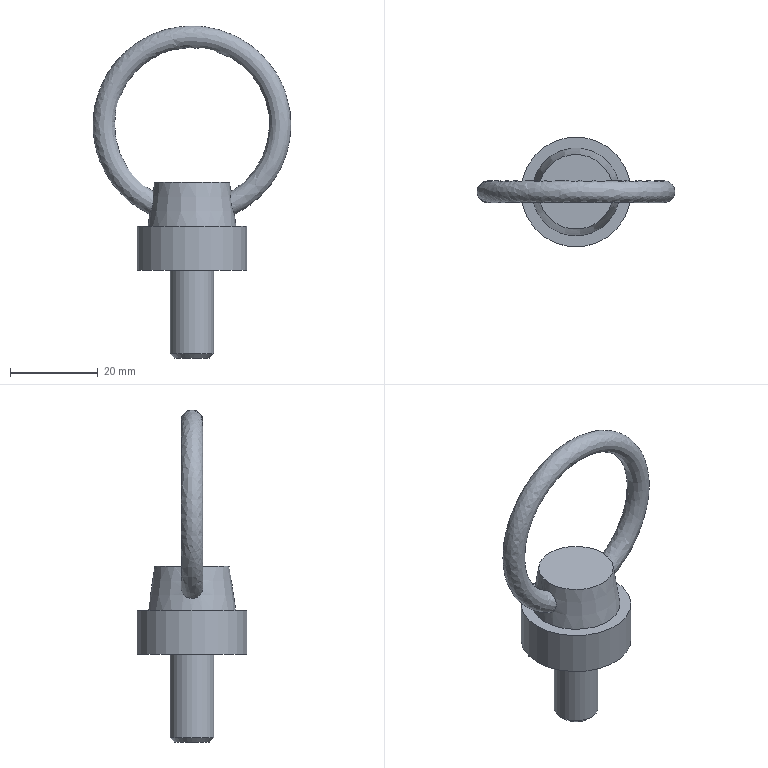Component | NX | LIFTING_EYE_M10 | 1 solid | 9 faces | volume 11253 mm3 | plane 4 | cone 2 | cylinder 2 | spline 1 | commonest cylinder face diameters 10 x1 25 x1